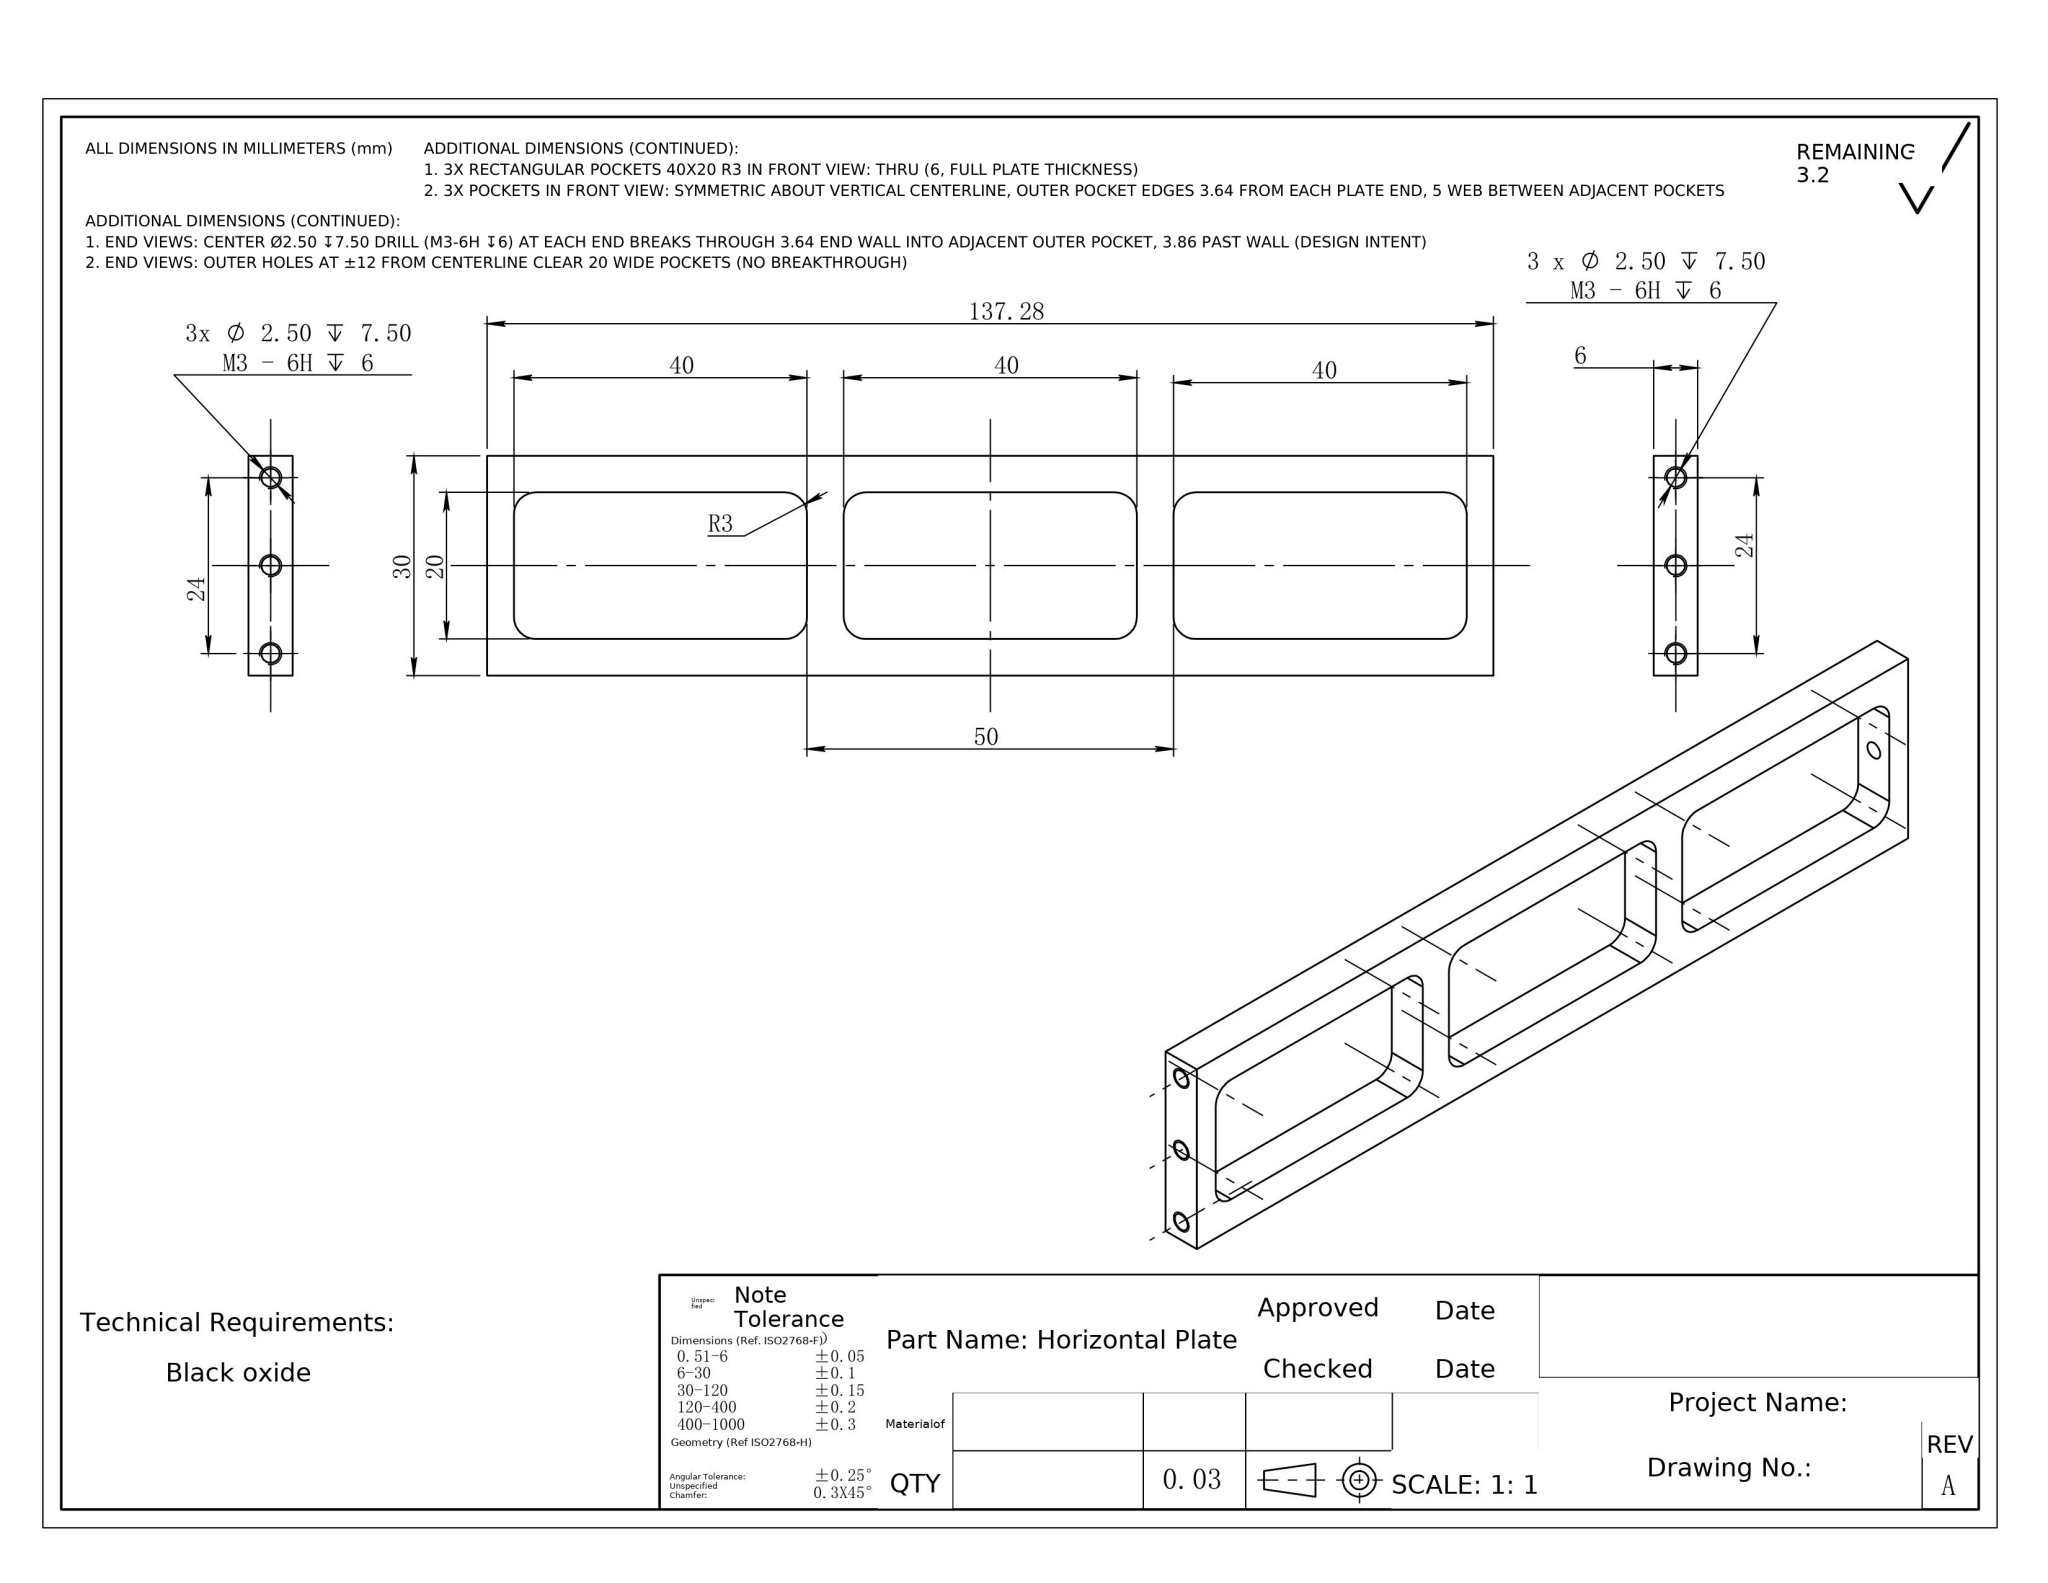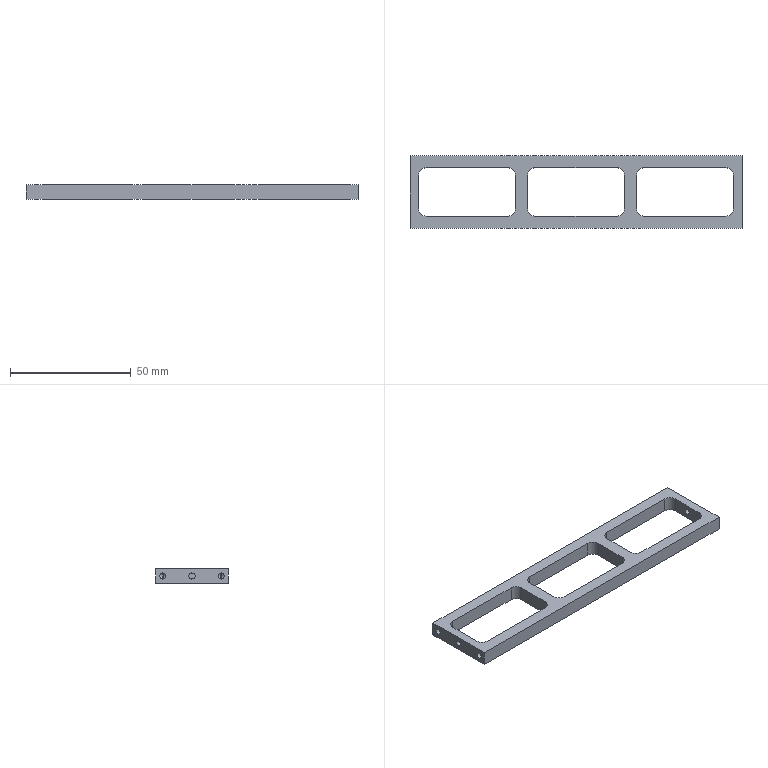Part | NX | mm | 1 solid | 50 faces | box 137.28 x 30 x 6 mm | volume 10262 mm3 | cylinder 24 | plane 18 | cone 8 | commonest cylinder face diameters 2.5 x12 6 x12